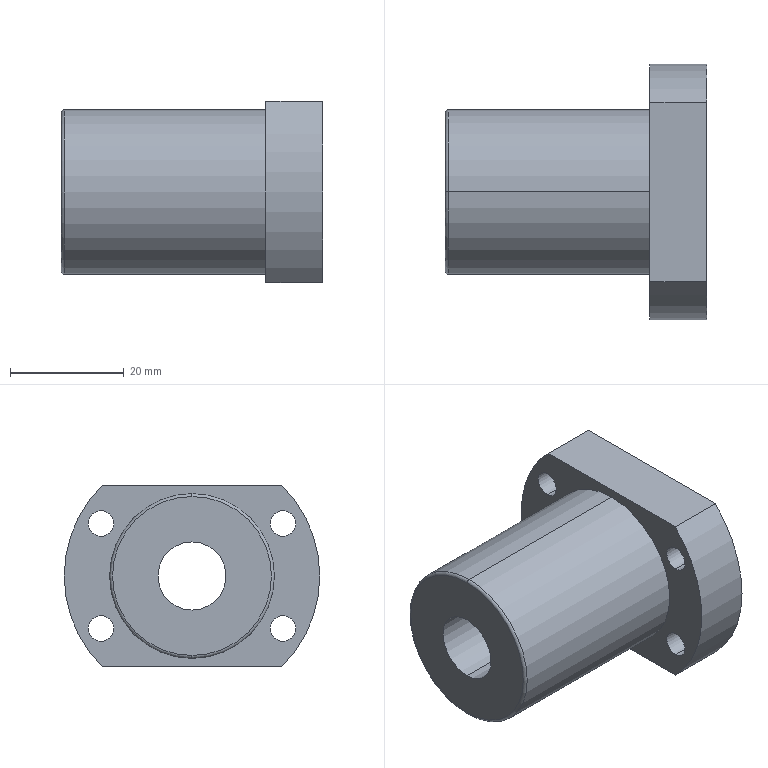Component | SolidWorks | BNK1208-2-Nut-1 | 1 solid | 21 faces | box 46 x 45 x 32 mm | volume 31007 mm3 | cylinder 14 | plane 5 | torus 2 | commonest cylinder face diameters 4.5 x8 12 x2 29 x2 45 x2
STEP:
#1=COLOUR_RGB('',0.7922,0.8196,0.9333);
#2=FILL_AREA_STYLE_COLOUR('',#1);
#3=FILL_AREA_STYLE('',(#2));
#4=SURFACE_STYLE_FILL_AREA(#3);
#5=SURFACE_SIDE_STYLE('',(#4));
#6=SURFACE_STYLE_USAGE(.BOTH.,#5);
#7=PRESENTATION_STYLE_ASSIGNMENT((#6));
#8=CARTESIAN_POINT('',(-2.212,0.7853,-0.4311));
#9=VERTEX_POINT('',#8);
#10=CARTESIAN_POINT('',(-2.212,0.7853,0.7107));
#11=VERTEX_POINT('',#10);
#12=CARTESIAN_POINT('',(-2.212,0.7853,0.1398));
#13=DIRECTION('',(1.,-0.,0.));
#14=DIRECTION('',(0.,0.,1.));
#15=AXIS2_PLACEMENT_3D('',#12,#13,#14);
#16=CIRCLE('',#15,0.5709);
#17=EDGE_CURVE('',#9,#11,#16,.T.);
#18=ORIENTED_EDGE('',*,*,#17,.F.);
#19=CARTESIAN_POINT('',(-2.232,0.7853,-0.4114));
#20=VERTEX_POINT('',#19);
#21=CARTESIAN_POINT('',(-2.212,0.7853,-0.4114));
#22=DIRECTION('',(0.,1.,-0.));
#23=DIRECTION('',(0.,0.,1.));
#24=AXIS2_PLACEMENT_3D('',#21,#22,#23);
#25=CIRCLE('',#24,0.01969);
#26=EDGE_CURVE('',#9,#20,#25,.T.);
#27=ORIENTED_EDGE('',*,*,#26,.T.);
#28=CARTESIAN_POINT('',(-2.232,0.7853,0.691));
#29=VERTEX_POINT('',#28);
#30=CARTESIAN_POINT('',(-2.232,0.7853,0.1398));
#31=DIRECTION('',(-1.,0.,-0.));
#32=DIRECTION('',(0.,0.,1.));
#33=AXIS2_PLACEMENT_3D('',#30,#31,#32);
#34=CIRCLE('',#33,0.5512);
#35=EDGE_CURVE('',#29,#20,#34,.T.);
#36=ORIENTED_EDGE('',*,*,#35,.F.);
#37=CARTESIAN_POINT('',(-2.212,0.7853,0.691));
#38=DIRECTION('',(-0.,-1.,0.));
#39=DIRECTION('',(0.,0.,-1.));
#40=AXIS2_PLACEMENT_3D('',#37,#38,#39);
#41=CIRCLE('',#40,0.01969);
#42=EDGE_CURVE('',#11,#29,#41,.T.);
#43=ORIENTED_EDGE('',*,*,#42,.F.);
#44=EDGE_LOOP('',(#18,#27,#36,#43));
#45=FACE_OUTER_BOUND('',#44,.T.);
#46=CARTESIAN_POINT('',(-2.212,0.7853,0.1398));
#47=DIRECTION('',(-1.,0.,-0.));
#48=DIRECTION('',(-0.,0.,1.));
#49=AXIS2_PLACEMENT_3D('',#46,#47,#48);
#50=TOROIDAL_SURFACE('',#49,0.5512,0.01969);
#51=ADVANCED_FACE('',(#45),#50,.T.);
#52=CARTESIAN_POINT('',(-0.8147,1.416,-0.1358));
#53=VERTEX_POINT('',#52);
#54=CARTESIAN_POINT('',(-0.8147,1.416,-0.313));
#55=VERTEX_POINT('',#54);
#56=CARTESIAN_POINT('',(-0.8147,1.416,-0.2244));
#57=DIRECTION('',(1.,-0.,0.));
#58=DIRECTION('',(0.,0.,-1.));
#59=AXIS2_PLACEMENT_3D('',#56,#57,#58);
#60=CIRCLE('',#59,0.08858);
#61=EDGE_CURVE('',#53,#55,#60,.T.);
#62=ORIENTED_EDGE('',*,*,#61,.F.);
#63=CARTESIAN_POINT('',(-0.421,1.416,-0.1358));
#64=VERTEX_POINT('',#63);
#65=CARTESIAN_POINT('',(-0.421,1.416,-0.1358));
#66=DIRECTION('',(1.,-0.,0.));
#67=VECTOR('',#66,39.37);
#68=LINE('',#65,#67);
#69=EDGE_CURVE('',#53,#64,#68,.T.);
#70=ORIENTED_EDGE('',*,*,#69,.T.);
#71=CARTESIAN_POINT('',(-0.421,1.416,-0.313));
#72=VERTEX_POINT('',#71);
#73=CARTESIAN_POINT('',(-0.421,1.416,-0.2244));
#74=DIRECTION('',(1.,-0.,0.));
#75=DIRECTION('',(0.,0.,-1.));
#76=AXIS2_PLACEMENT_3D('',#73,#74,#75);
#77=CIRCLE('',#76,0.08858);
#78=EDGE_CURVE('',#64,#72,#77,.T.);
#79=ORIENTED_EDGE('',*,*,#78,.T.);
#80=CARTESIAN_POINT('',(-0.421,1.416,-0.313));
#81=DIRECTION('',(1.,-0.,0.));
#82=VECTOR('',#81,39.37);
#83=LINE('',#80,#82);
#84=EDGE_CURVE('',#55,#72,#83,.T.);
#85=ORIENTED_EDGE('',*,*,#84,.F.);
#86=EDGE_LOOP('',(#62,#70,#79,#85));
#87=FACE_OUTER_BOUND('',#86,.T.);
#88=CARTESIAN_POINT('',(-0.421,1.416,-0.2244));
#89=DIRECTION('',(1.,-0.,0.));
#90=DIRECTION('',(0.,0.,-1.));
#91=AXIS2_PLACEMENT_3D('',#88,#89,#90);
#92=CYLINDRICAL_SURFACE('',#91,0.08858);
#93=ADVANCED_FACE('',(#87),#92,.F.);
#94=CARTESIAN_POINT('',(-0.8147,1.416,0.5925));
#95=VERTEX_POINT('',#94);
#96=CARTESIAN_POINT('',(-0.8147,1.416,0.4154));
#97=VERTEX_POINT('',#96);
#98=CARTESIAN_POINT('',(-0.8147,1.416,0.504));
#99=DIRECTION('',(1.,-0.,0.));
#100=DIRECTION('',(0.,0.,-1.));
#101=AXIS2_PLACEMENT_3D('',#98,#99,#100);
#102=CIRCLE('',#101,0.08858);
#103=EDGE_CURVE('',#95,#97,#102,.T.);
#104=ORIENTED_EDGE('',*,*,#103,.F.);
#105=CARTESIAN_POINT('',(-0.421,1.416,0.5925));
#106=VERTEX_POINT('',#105);
#107=CARTESIAN_POINT('',(-0.421,1.416,0.5925));
#108=DIRECTION('',(1.,-0.,0.));
#109=VECTOR('',#108,39.37);
#110=LINE('',#107,#109);
#111=EDGE_CURVE('',#95,#106,#110,.T.);
#112=ORIENTED_EDGE('',*,*,#111,.T.);
#113=CARTESIAN_POINT('',(-0.421,1.416,0.4154));
#114=VERTEX_POINT('',#113);
#115=CARTESIAN_POINT('',(-0.421,1.416,0.504));
#116=DIRECTION('',(1.,-0.,0.));
#117=DIRECTION('',(0.,0.,-1.));
#118=AXIS2_PLACEMENT_3D('',#115,#116,#117);
#119=CIRCLE('',#118,0.08858);
#120=EDGE_CURVE('',#106,#114,#119,.T.);
#121=ORIENTED_EDGE('',*,*,#120,.T.);
#122=CARTESIAN_POINT('',(-0.421,1.416,0.4154));
#123=DIRECTION('',(1.,-0.,0.));
#124=VECTOR('',#123,39.37);
#125=LINE('',#122,#124);
#126=EDGE_CURVE('',#97,#114,#125,.T.);
#127=ORIENTED_EDGE('',*,*,#126,.F.);
#128=EDGE_LOOP('',(#104,#112,#121,#127));
#129=FACE_OUTER_BOUND('',#128,.T.);
#130=CARTESIAN_POINT('',(-0.421,1.416,0.504));
#131=DIRECTION('',(1.,-0.,0.));
#132=DIRECTION('',(0.,0.,-1.));
#133=AXIS2_PLACEMENT_3D('',#130,#131,#132);
#134=CYLINDRICAL_SURFACE('',#133,0.08858);
#135=ADVANCED_FACE('',(#129),#134,.F.);
#136=CARTESIAN_POINT('',(-0.8147,0.1545,0.5925));
#137=VERTEX_POINT('',#136);
#138=CARTESIAN_POINT('',(-0.8147,0.1545,0.4154));
#139=VERTEX_POINT('',#138);
#140=CARTESIAN_POINT('',(-0.8147,0.1545,0.504));
#141=DIRECTION('',(1.,-0.,0.));
#142=DIRECTION('',(0.,-0.,-1.));
#143=AXIS2_PLACEMENT_3D('',#140,#141,#142);
#144=CIRCLE('',#143,0.08858);
#145=EDGE_CURVE('',#137,#139,#144,.T.);
#146=ORIENTED_EDGE('',*,*,#145,.F.);
#147=CARTESIAN_POINT('',(-0.421,0.1545,0.5925));
#148=VERTEX_POINT('',#147);
#149=CARTESIAN_POINT('',(-0.421,0.1545,0.5925));
#150=DIRECTION('',(1.,-0.,0.));
#151=VECTOR('',#150,39.37);
#152=LINE('',#149,#151);
#153=EDGE_CURVE('',#137,#148,#152,.T.);
#154=ORIENTED_EDGE('',*,*,#153,.T.);
#155=CARTESIAN_POINT('',(-0.421,0.1545,0.4154));
#156=VERTEX_POINT('',#155);
#157=CARTESIAN_POINT('',(-0.421,0.1545,0.504));
#158=DIRECTION('',(1.,-0.,0.));
#159=DIRECTION('',(0.,-0.,-1.));
#160=AXIS2_PLACEMENT_3D('',#157,#158,#159);
#161=CIRCLE('',#160,0.08858);
#162=EDGE_CURVE('',#148,#156,#161,.T.);
#163=ORIENTED_EDGE('',*,*,#162,.T.);
#164=CARTESIAN_POINT('',(-0.421,0.1545,0.4154));
#165=DIRECTION('',(1.,-0.,0.));
#166=VECTOR('',#165,39.37);
#167=LINE('',#164,#166);
#168=EDGE_CURVE('',#139,#156,#167,.T.);
#169=ORIENTED_EDGE('',*,*,#168,.F.);
#170=EDGE_LOOP('',(#146,#154,#163,#169));
#171=FACE_OUTER_BOUND('',#170,.T.);
#172=CARTESIAN_POINT('',(-0.421,0.1545,0.504));
#173=DIRECTION('',(1.,-0.,0.));
#174=DIRECTION('',(0.,-0.,-1.));
#175=AXIS2_PLACEMENT_3D('',#172,#173,#174);
#176=CYLINDRICAL_SURFACE('',#175,0.08858);
#177=ADVANCED_FACE('',(#171),#176,.F.);
#178=CARTESIAN_POINT('',(-0.8147,0.1545,-0.1358));
#179=VERTEX_POINT('',#178);
#180=CARTESIAN_POINT('',(-0.8147,0.1545,-0.313));
#181=VERTEX_POINT('',#180);
#182=CARTESIAN_POINT('',(-0.8147,0.1545,-0.2244));
#183=DIRECTION('',(1.,-0.,0.));
#184=DIRECTION('',(0.,-0.,-1.));
#185=AXIS2_PLACEMENT_3D('',#182,#183,#184);
#186=CIRCLE('',#185,0.08858);
#187=EDGE_CURVE('',#179,#181,#186,.T.);
#188=ORIENTED_EDGE('',*,*,#187,.F.);
#189=CARTESIAN_POINT('',(-0.421,0.1545,-0.1358));
#190=VERTEX_POINT('',#189);
#191=CARTESIAN_POINT('',(-0.421,0.1545,-0.1358));
#192=DIRECTION('',(1.,-0.,0.));
#193=VECTOR('',#192,39.37);
#194=LINE('',#191,#193);
#195=EDGE_CURVE('',#179,#190,#194,.T.);
#196=ORIENTED_EDGE('',*,*,#195,.T.);
#197=CARTESIAN_POINT('',(-0.421,0.1545,-0.313));
#198=VERTEX_POINT('',#197);
#199=CARTESIAN_POINT('',(-0.421,0.1545,-0.2244));
#200=DIRECTION('',(1.,-0.,0.));
#201=DIRECTION('',(0.,-0.,-1.));
#202=AXIS2_PLACEMENT_3D('',#199,#200,#201);
#203=CIRCLE('',#202,0.08858);
#204=EDGE_CURVE('',#190,#198,#203,.T.);
#205=ORIENTED_EDGE('',*,*,#204,.T.);
#206=CARTESIAN_POINT('',(-0.421,0.1545,-0.313));
#207=DIRECTION('',(1.,-0.,0.));
#208=VECTOR('',#207,39.37);
#209=LINE('',#206,#208);
#210=EDGE_CURVE('',#181,#198,#209,.T.);
#211=ORIENTED_EDGE('',*,*,#210,.F.);
#212=EDGE_LOOP('',(#188,#196,#205,#211));
#213=FACE_OUTER_BOUND('',#212,.T.);
#214=CARTESIAN_POINT('',(-0.421,0.1545,-0.2244));
#215=DIRECTION('',(1.,-0.,0.));
#216=DIRECTION('',(0.,-0.,-1.));
#217=AXIS2_PLACEMENT_3D('',#214,#215,#216);
#218=CYLINDRICAL_SURFACE('',#217,0.08858);
#219=ADVANCED_FACE('',(#213),#218,.F.);
#220=CARTESIAN_POINT('',(-2.232,0.7853,-0.09643));
#221=VERTEX_POINT('',#220);
#222=CARTESIAN_POINT('',(-2.232,0.7853,0.376));
#223=VERTEX_POINT('',#222);
#224=CARTESIAN_POINT('',(-2.232,0.7853,0.1398));
#225=DIRECTION('',(-1.,0.,-0.));
#226=DIRECTION('',(0.,0.,1.));
#227=AXIS2_PLACEMENT_3D('',#224,#225,#226);
#228=CIRCLE('',#227,0.2362);
#229=EDGE_CURVE('',#221,#223,#228,.T.);
#230=ORIENTED_EDGE('',*,*,#229,.T.);
#231=CARTESIAN_POINT('',(-0.421,0.7853,0.376));
#232=VERTEX_POINT('',#231);
#233=CARTESIAN_POINT('',(-2.39,0.7853,0.376));
#234=DIRECTION('',(1.,-0.,0.));
#235=VECTOR('',#234,39.37);
#236=LINE('',#233,#235);
#237=EDGE_CURVE('',#223,#232,#236,.T.);
#238=ORIENTED_EDGE('',*,*,#237,.T.);
#239=CARTESIAN_POINT('',(-0.421,0.7853,-0.09643));
#240=VERTEX_POINT('',#239);
#241=CARTESIAN_POINT('',(-0.421,0.7853,0.1398));
#242=DIRECTION('',(1.,-0.,0.));
#243=DIRECTION('',(0.,-0.,-1.));
#244=AXIS2_PLACEMENT_3D('',#241,#242,#243);
#245=CIRCLE('',#244,0.2362);
#246=EDGE_CURVE('',#232,#240,#245,.T.);
#247=ORIENTED_EDGE('',*,*,#246,.T.);
#248=CARTESIAN_POINT('',(-2.39,0.7853,-0.09643));
#249=DIRECTION('',(1.,-0.,0.));
#250=VECTOR('',#249,39.37);
#251=LINE('',#248,#250);
#252=EDGE_CURVE('',#221,#240,#251,.T.);
#253=ORIENTED_EDGE('',*,*,#252,.F.);
#254=EDGE_LOOP('',(#230,#238,#247,#253));
#255=FACE_OUTER_BOUND('',#254,.T.);
#256=CARTESIAN_POINT('',(-2.39,0.7853,0.1398));
#257=DIRECTION('',(1.,-0.,0.));
#258=DIRECTION('',(0.,-0.,-1.));
#259=AXIS2_PLACEMENT_3D('',#256,#257,#258);
#260=CYLINDRICAL_SURFACE('',#259,0.2362);
#261=ADVANCED_FACE('',(#255),#260,.F.);
#262=ORIENTED_EDGE('',*,*,#17,.T.);
#263=CARTESIAN_POINT('',(-0.8147,0.7853,0.7107));
#264=VERTEX_POINT('',#263);
#265=CARTESIAN_POINT('',(-2.232,0.7853,0.7107));
#266=DIRECTION('',(1.,-0.,0.));
#267=VECTOR('',#266,39.37);
#268=LINE('',#265,#267);
#269=EDGE_CURVE('',#11,#264,#268,.T.);
#270=ORIENTED_EDGE('',*,*,#269,.T.);
#271=CARTESIAN_POINT('',(-0.8147,0.7853,-0.4311));
#272=VERTEX_POINT('',#271);
#273=CARTESIAN_POINT('',(-0.8147,0.7853,0.1398));
#274=DIRECTION('',(1.,-0.,0.));
#275=DIRECTION('',(0.,-0.,-1.));
#276=AXIS2_PLACEMENT_3D('',#273,#274,#275);
#277=CIRCLE('',#276,0.5709);
#278=EDGE_CURVE('',#272,#264,#277,.T.);
#279=ORIENTED_EDGE('',*,*,#278,.F.);
#280=CARTESIAN_POINT('',(-2.232,0.7853,-0.4311));
#281=DIRECTION('',(1.,-0.,0.));
#282=VECTOR('',#281,39.37);
#283=LINE('',#280,#282);
#284=EDGE_CURVE('',#9,#272,#283,.T.);
#285=ORIENTED_EDGE('',*,*,#284,.F.);
#286=EDGE_LOOP('',(#262,#270,#279,#285));
#287=FACE_OUTER_BOUND('',#286,.T.);
#288=CARTESIAN_POINT('',(-2.232,0.7853,0.1398));
#289=DIRECTION('',(1.,-0.,0.));
#290=DIRECTION('',(0.,-0.,-1.));
#291=AXIS2_PLACEMENT_3D('',#288,#289,#290);
#292=CYLINDRICAL_SURFACE('',#291,0.5709);
#293=ADVANCED_FACE('',(#287),#292,.T.);
#294=CARTESIAN_POINT('',(-0.421,0.1624,0.7697));
#295=VERTEX_POINT('',#294);
#296=CARTESIAN_POINT('',(-0.421,0.1624,-0.4901));
#297=VERTEX_POINT('',#296);
#298=CARTESIAN_POINT('',(-0.421,0.7853,0.1398));
#299=DIRECTION('',(1.,-0.,0.));
#300=DIRECTION('',(0.,-0.,-1.));
#301=AXIS2_PLACEMENT_3D('',#298,#299,#300);
#302=CIRCLE('',#301,0.8858);
#303=EDGE_CURVE('',#295,#297,#302,.T.);
#304=ORIENTED_EDGE('',*,*,#303,.F.);
#305=CARTESIAN_POINT('',(-0.8147,0.1624,0.7697));
#306=VERTEX_POINT('',#305);
#307=CARTESIAN_POINT('',(-2.39,0.1624,0.7697));
#308=DIRECTION('',(1.,-0.,0.));
#309=VECTOR('',#308,39.37);
#310=LINE('',#307,#309);
#311=EDGE_CURVE('',#306,#295,#310,.T.);
#312=ORIENTED_EDGE('',*,*,#311,.F.);
#313=CARTESIAN_POINT('',(-0.8147,0.1624,-0.4901));
#314=VERTEX_POINT('',#313);
#315=CARTESIAN_POINT('',(-0.8147,0.7853,0.1398));
#316=DIRECTION('',(1.,-0.,0.));
#317=DIRECTION('',(0.,-0.,-1.));
#318=AXIS2_PLACEMENT_3D('',#315,#316,#317);
#319=CIRCLE('',#318,0.8858);
#320=EDGE_CURVE('',#306,#314,#319,.T.);
#321=ORIENTED_EDGE('',*,*,#320,.T.);
#322=CARTESIAN_POINT('',(-2.39,0.1624,-0.4901));
#323=DIRECTION('',(1.,-0.,0.));
#324=VECTOR('',#323,39.37);
#325=LINE('',#322,#324);
#326=EDGE_CURVE('',#314,#297,#325,.T.);
#327=ORIENTED_EDGE('',*,*,#326,.T.);
#328=EDGE_LOOP('',(#304,#312,#321,#327));
#329=FACE_OUTER_BOUND('',#328,.T.);
#330=CARTESIAN_POINT('',(-0.421,0.7853,0.1398));
#331=DIRECTION('',(-1.,0.,-0.));
#332=DIRECTION('',(0.,0.,1.));
#333=AXIS2_PLACEMENT_3D('',#330,#331,#332);
#334=CYLINDRICAL_SURFACE('',#333,0.8858);
#335=ADVANCED_FACE('',(#329),#334,.T.);
#336=ORIENTED_EDGE('',*,*,#269,.F.);
#337=CARTESIAN_POINT('',(-2.212,0.7853,0.1398));
#338=DIRECTION('',(1.,-0.,0.));
#339=DIRECTION('',(0.,0.,1.));
#340=AXIS2_PLACEMENT_3D('',#337,#338,#339);
#341=CIRCLE('',#340,0.5709);
#342=EDGE_CURVE('',#11,#9,#341,.T.);
#343=ORIENTED_EDGE('',*,*,#342,.T.);
#344=ORIENTED_EDGE('',*,*,#284,.T.);
#345=CARTESIAN_POINT('',(-0.8147,0.7853,0.1398));
#346=DIRECTION('',(1.,-0.,0.));
#347=DIRECTION('',(0.,-0.,-1.));
#348=AXIS2_PLACEMENT_3D('',#345,#346,#347);
#349=CIRCLE('',#348,0.5709);
#350=EDGE_CURVE('',#264,#272,#349,.T.);
#351=ORIENTED_EDGE('',*,*,#350,.F.);
#352=EDGE_LOOP('',(#336,#343,#344,#351));
#353=FACE_OUTER_BOUND('',#352,.T.);
#354=CARTESIAN_POINT('',(-2.232,0.7853,0.1398));
#355=DIRECTION('',(1.,-0.,0.));
#356=DIRECTION('',(0.,-0.,-1.));
#357=AXIS2_PLACEMENT_3D('',#354,#355,#356);
#358=CYLINDRICAL_SURFACE('',#357,0.5709);
#359=ADVANCED_FACE('',(#353),#358,.T.);
#360=ORIENTED_EDGE('',*,*,#35,.T.);
#361=CARTESIAN_POINT('',(-2.232,0.7853,0.1398));
#362=DIRECTION('',(-1.,0.,-0.));
#363=DIRECTION('',(0.,0.,1.));
#364=AXIS2_PLACEMENT_3D('',#361,#362,#363);
#365=CIRCLE('',#364,0.5512);
#366=EDGE_CURVE('',#20,#29,#365,.T.);
#367=ORIENTED_EDGE('',*,*,#366,.T.);
#368=EDGE_LOOP('',(#360,#367));
#369=FACE_OUTER_BOUND('',#368,.T.);
#370=ORIENTED_EDGE('',*,*,#229,.F.);
#371=CARTESIAN_POINT('',(-2.232,0.7853,0.1398));
#372=DIRECTION('',(-1.,0.,-0.));
#373=DIRECTION('',(0.,0.,1.));
#374=AXIS2_PLACEMENT_3D('',#371,#372,#373);
#375=CIRCLE('',#374,0.2362);
#376=EDGE_CURVE('',#223,#221,#375,.T.);
#377=ORIENTED_EDGE('',*,*,#376,.F.);
#378=EDGE_LOOP('',(#370,#377));
#379=FACE_BOUND('',#378,.T.);
#380=CARTESIAN_POINT('',(-2.232,0.7853,0.1398));
#381=DIRECTION('',(-1.,0.,-0.));
#382=DIRECTION('',(-0.,0.,1.));
#383=AXIS2_PLACEMENT_3D('',#380,#381,#382);
#384=PLANE('',#383);
#385=ADVANCED_FACE('',(#369,#379),#384,.T.);
#386=CARTESIAN_POINT('',(-0.8147,1.416,-0.2244));
#387=DIRECTION('',(1.,-0.,0.));
#388=DIRECTION('',(0.,0.,-1.));
#389=AXIS2_PLACEMENT_3D('',#386,#387,#388);
#390=CIRCLE('',#389,0.08858);
#391=EDGE_CURVE('',#55,#53,#390,.T.);
#392=ORIENTED_EDGE('',*,*,#391,.T.);
#393=ORIENTED_EDGE('',*,*,#61,.T.);
#394=EDGE_LOOP('',(#392,#393));
#395=FACE_BOUND('',#394,.T.);
#396=CARTESIAN_POINT('',(-0.8147,1.416,0.504));
#397=DIRECTION('',(1.,-0.,0.));
#398=DIRECTION('',(0.,0.,-1.));
#399=AXIS2_PLACEMENT_3D('',#396,#397,#398);
#400=CIRCLE('',#399,0.08858);
#401=EDGE_CURVE('',#97,#95,#400,.T.);
#402=ORIENTED_EDGE('',*,*,#401,.T.);
#403=ORIENTED_EDGE('',*,*,#103,.T.);
#404=EDGE_LOOP('',(#402,#403));
#405=FACE_BOUND('',#404,.T.);
#406=CARTESIAN_POINT('',(-0.8147,0.1545,0.504));
#407=DIRECTION('',(1.,-0.,0.));
#408=DIRECTION('',(0.,-0.,-1.));
#409=AXIS2_PLACEMENT_3D('',#406,#407,#408);
#410=CIRCLE('',#409,0.08858);
#411=EDGE_CURVE('',#139,#137,#410,.T.);
#412=ORIENTED_EDGE('',*,*,#411,.T.);
#413=ORIENTED_EDGE('',*,*,#145,.T.);
#414=EDGE_LOOP('',(#412,#413));
#415=FACE_BOUND('',#414,.T.);
#416=CARTESIAN_POINT('',(-0.8147,0.1545,-0.2244));
#417=DIRECTION('',(1.,-0.,0.));
#418=DIRECTION('',(0.,-0.,-1.));
#419=AXIS2_PLACEMENT_3D('',#416,#417,#418);
#420=CIRCLE('',#419,0.08858);
#421=EDGE_CURVE('',#181,#179,#420,.T.);
#422=ORIENTED_EDGE('',*,*,#421,.T.);
#423=ORIENTED_EDGE('',*,*,#187,.T.);
#424=EDGE_LOOP('',(#422,#423));
#425=FACE_BOUND('',#424,.T.);
#426=ORIENTED_EDGE('',*,*,#320,.F.);
#427=CARTESIAN_POINT('',(-0.8147,1.408,0.7697));
#428=VERTEX_POINT('',#427);
#429=CARTESIAN_POINT('',(-0.8147,0.7853,0.7697));
#430=DIRECTION('',(0.,1.,-0.));
#431=VECTOR('',#430,39.37);
#432=LINE('',#429,#431);
#433=EDGE_CURVE('',#306,#428,#432,.T.);
#434=ORIENTED_EDGE('',*,*,#433,.T.);
#435=CARTESIAN_POINT('',(-0.8147,1.408,-0.4901));
#436=VERTEX_POINT('',#435);
#437=CARTESIAN_POINT('',(-0.8147,0.7853,0.1398));
#438=DIRECTION('',(1.,-0.,0.));
#439=DIRECTION('',(0.,-0.,-1.));
#440=AXIS2_PLACEMENT_3D('',#437,#438,#439);
#441=CIRCLE('',#440,0.8858);
#442=EDGE_CURVE('',#436,#428,#441,.T.);
#443=ORIENTED_EDGE('',*,*,#442,.F.);
#444=CARTESIAN_POINT('',(-0.8147,0.7853,-0.4901));
#445=DIRECTION('',(-0.,-1.,0.));
#446=VECTOR('',#445,39.37);
#447=LINE('',#444,#446);
#448=EDGE_CURVE('',#436,#314,#447,.T.);
#449=ORIENTED_EDGE('',*,*,#448,.T.);
#450=EDGE_LOOP('',(#426,#434,#443,#449));
#451=FACE_OUTER_BOUND('',#450,.T.);
#452=ORIENTED_EDGE('',*,*,#278,.T.);
#453=ORIENTED_EDGE('',*,*,#350,.T.);
#454=EDGE_LOOP('',(#452,#453));
#455=FACE_BOUND('',#454,.T.);
#456=CARTESIAN_POINT('',(-0.8147,0.7853,0.1398));
#457=DIRECTION('',(1.,-0.,0.));
#458=DIRECTION('',(0.,-0.,-1.));
#459=AXIS2_PLACEMENT_3D('',#456,#457,#458);
#460=PLANE('',#459);
#461=ADVANCED_FACE('',(#395,#405,#415,#425,#451,#455),#460,.F.);
#462=ORIENTED_EDGE('',*,*,#442,.T.);
#463=CARTESIAN_POINT('',(-0.421,1.408,0.7697));
#464=VERTEX_POINT('',#463);
#465=CARTESIAN_POINT('',(-2.39,1.408,0.7697));
#466=DIRECTION('',(1.,-0.,0.));
#467=VECTOR('',#466,39.37);
#468=LINE('',#465,#467);
#469=EDGE_CURVE('',#428,#464,#468,.T.);
#470=ORIENTED_EDGE('',*,*,#469,.T.);
#471=CARTESIAN_POINT('',(-0.421,1.408,-0.4901));
#472=VERTEX_POINT('',#471);
#473=CARTESIAN_POINT('',(-0.421,0.7853,0.1398));
#474=DIRECTION('',(1.,-0.,0.));
#475=DIRECTION('',(0.,-0.,-1.));
#476=AXIS2_PLACEMENT_3D('',#473,#474,#475);
#477=CIRCLE('',#476,0.8858);
#478=EDGE_CURVE('',#472,#464,#477,.T.);
#479=ORIENTED_EDGE('',*,*,#478,.F.);
#480=CARTESIAN_POINT('',(-2.39,1.408,-0.4901));
#481=DIRECTION('',(1.,-0.,0.));
#482=VECTOR('',#481,39.37);
#483=LINE('',#480,#482);
#484=EDGE_CURVE('',#436,#472,#483,.T.);
#485=ORIENTED_EDGE('',*,*,#484,.F.);
#486=EDGE_LOOP('',(#462,#470,#479,#485));
#487=FACE_OUTER_BOUND('',#486,.T.);
#488=CARTESIAN_POINT('',(-0.421,0.7853,0.1398));
#489=DIRECTION('',(-1.,0.,-0.));
#490=DIRECTION('',(0.,0.,1.));
#491=AXIS2_PLACEMENT_3D('',#488,#489,#490);
#492=CYLINDRICAL_SURFACE('',#491,0.8858);
#493=ADVANCED_FACE('',(#487),#492,.T.);
#494=CARTESIAN_POINT('',(-0.421,1.416,-0.2244));
#495=DIRECTION('',(1.,-0.,0.));
#496=DIRECTION('',(0.,0.,-1.));
#497=AXIS2_PLACEMENT_3D('',#494,#495,#496);
#498=CIRCLE('',#497,0.08858);
#499=EDGE_CURVE('',#72,#64,#498,.T.);
#500=ORIENTED_EDGE('',*,*,#499,.F.);
#501=ORIENTED_EDGE('',*,*,#78,.F.);
#502=EDGE_LOOP('',(#500,#501));
#503=FACE_BOUND('',#502,.T.);
#504=CARTESIAN_POINT('',(-0.421,1.416,0.504));
#505=DIRECTION('',(1.,-0.,0.));
#506=DIRECTION('',(0.,0.,-1.));
#507=AXIS2_PLACEMENT_3D('',#504,#505,#506);
#508=CIRCLE('',#507,0.08858);
#509=EDGE_CURVE('',#114,#106,#508,.T.);
#510=ORIENTED_EDGE('',*,*,#509,.F.);
#511=ORIENTED_EDGE('',*,*,#120,.F.);
#512=EDGE_LOOP('',(#510,#511));
#513=FACE_BOUND('',#512,.T.);
#514=CARTESIAN_POINT('',(-0.421,0.1545,0.504));
#515=DIRECTION('',(1.,-0.,0.));
#516=DIRECTION('',(0.,-0.,-1.));
#517=AXIS2_PLACEMENT_3D('',#514,#515,#516);
#518=CIRCLE('',#517,0.08858);
#519=EDGE_CURVE('',#156,#148,#518,.T.);
#520=ORIENTED_EDGE('',*,*,#519,.F.);
#521=ORIENTED_EDGE('',*,*,#162,.F.);
#522=EDGE_LOOP('',(#520,#521));
#523=FACE_BOUND('',#522,.T.);
#524=CARTESIAN_POINT('',(-0.421,0.1545,-0.2244));
#525=DIRECTION('',(1.,-0.,0.));
#526=DIRECTION('',(0.,-0.,-1.));
#527=AXIS2_PLACEMENT_3D('',#524,#525,#526);
#528=CIRCLE('',#527,0.08858);
#529=EDGE_CURVE('',#198,#190,#528,.T.);
#530=ORIENTED_EDGE('',*,*,#529,.F.);
#531=ORIENTED_EDGE('',*,*,#204,.F.);
#532=EDGE_LOOP('',(#530,#531));
#533=FACE_BOUND('',#532,.T.);
#534=CARTESIAN_POINT('',(-0.421,0.7853,0.1398));
#535=DIRECTION('',(1.,-0.,0.));
#536=DIRECTION('',(0.,-0.,-1.));
#537=AXIS2_PLACEMENT_3D('',#534,#535,#536);
#538=CIRCLE('',#537,0.2362);
#539=EDGE_CURVE('',#240,#232,#538,.T.);
#540=ORIENTED_EDGE('',*,*,#539,.F.);
#541=ORIENTED_EDGE('',*,*,#246,.F.);
#542=EDGE_LOOP('',(#540,#541));
#543=FACE_BOUND('',#542,.T.);
#544=CARTESIAN_POINT('',(-0.421,1.408,0.7697));
#545=DIRECTION('',(0.,1.,-0.));
#546=VECTOR('',#545,39.37);
#547=LINE('',#544,#546);
#548=EDGE_CURVE('',#295,#464,#547,.T.);
#549=ORIENTED_EDGE('',*,*,#548,.F.);
#550=ORIENTED_EDGE('',*,*,#303,.T.);
#551=CARTESIAN_POINT('',(-0.421,1.408,-0.4901));
#552=DIRECTION('',(-0.,-1.,0.));
#553=VECTOR('',#552,39.37);
#554=LINE('',#551,#553);
#555=EDGE_CURVE('',#472,#297,#554,.T.);
#556=ORIENTED_EDGE('',*,*,#555,.F.);
#557=ORIENTED_EDGE('',*,*,#478,.T.);
#558=EDGE_LOOP('',(#549,#550,#556,#557));
#559=FACE_OUTER_BOUND('',#558,.T.);
#560=CARTESIAN_POINT('',(-0.421,0.7853,0.1398));
#561=DIRECTION('',(1.,-0.,0.));
#562=DIRECTION('',(0.,-0.,-1.));
#563=AXIS2_PLACEMENT_3D('',#560,#561,#562);
#564=PLANE('',#563);
#565=ADVANCED_FACE('',(#503,#513,#523,#533,#543,#559),#564,.T.);
#566=ORIENTED_EDGE('',*,*,#484,.T.);
#567=ORIENTED_EDGE('',*,*,#555,.T.);
#568=ORIENTED_EDGE('',*,*,#326,.F.);
#569=ORIENTED_EDGE('',*,*,#448,.F.);
#570=EDGE_LOOP('',(#566,#567,#568,#569));
#571=FACE_OUTER_BOUND('',#570,.T.);
#572=CARTESIAN_POINT('',(-2.39,1.408,-0.4901));
#573=DIRECTION('',(-0.,0.,1.));
#574=DIRECTION('',(1.,-0.,0.));
#575=AXIS2_PLACEMENT_3D('',#572,#573,#574);
#576=PLANE('',#575);
#577=ADVANCED_FACE('',(#571),#576,.F.);
#578=ORIENTED_EDGE('',*,*,#311,.T.);
#579=ORIENTED_EDGE('',*,*,#548,.T.);
#580=ORIENTED_EDGE('',*,*,#469,.F.);
#581=ORIENTED_EDGE('',*,*,#433,.F.);
#582=EDGE_LOOP('',(#578,#579,#580,#581));
#583=FACE_OUTER_BOUND('',#582,.T.);
#584=CARTESIAN_POINT('',(-2.39,1.408,0.7697));
#585=DIRECTION('',(0.,-0.,-1.));
#586=DIRECTION('',(-1.,0.,-0.));
#587=AXIS2_PLACEMENT_3D('',#584,#585,#586);
#588=PLANE('',#587);
#589=ADVANCED_FACE('',(#583),#588,.F.);
#590=ORIENTED_EDGE('',*,*,#237,.F.);
#591=ORIENTED_EDGE('',*,*,#376,.T.);
#592=ORIENTED_EDGE('',*,*,#252,.T.);
#593=ORIENTED_EDGE('',*,*,#539,.T.);
#594=EDGE_LOOP('',(#590,#591,#592,#593));
#595=FACE_OUTER_BOUND('',#594,.T.);
#596=CARTESIAN_POINT('',(-2.39,0.7853,0.1398));
#597=DIRECTION('',(1.,-0.,0.));
#598=DIRECTION('',(0.,-0.,-1.));
#599=AXIS2_PLACEMENT_3D('',#596,#597,#598);
#600=CYLINDRICAL_SURFACE('',#599,0.2362);
#601=ADVANCED_FACE('',(#595),#600,.F.);
#602=ORIENTED_EDGE('',*,*,#195,.F.);
#603=ORIENTED_EDGE('',*,*,#421,.F.);
#604=ORIENTED_EDGE('',*,*,#210,.T.);
#605=ORIENTED_EDGE('',*,*,#529,.T.);
#606=EDGE_LOOP('',(#602,#603,#604,#605));
#607=FACE_OUTER_BOUND('',#606,.T.);
#608=CARTESIAN_POINT('',(-0.421,0.1545,-0.2244));
#609=DIRECTION('',(1.,-0.,0.));
#610=DIRECTION('',(0.,-0.,-1.));
#611=AXIS2_PLACEMENT_3D('',#608,#609,#610);
#612=CYLINDRICAL_SURFACE('',#611,0.08858);
#613=ADVANCED_FACE('',(#607),#612,.F.);
#614=ORIENTED_EDGE('',*,*,#153,.F.);
#615=ORIENTED_EDGE('',*,*,#411,.F.);
#616=ORIENTED_EDGE('',*,*,#168,.T.);
#617=ORIENTED_EDGE('',*,*,#519,.T.);
#618=EDGE_LOOP('',(#614,#615,#616,#617));
#619=FACE_OUTER_BOUND('',#618,.T.);
#620=CARTESIAN_POINT('',(-0.421,0.1545,0.504));
#621=DIRECTION('',(1.,-0.,0.));
#622=DIRECTION('',(0.,-0.,-1.));
#623=AXIS2_PLACEMENT_3D('',#620,#621,#622);
#624=CYLINDRICAL_SURFACE('',#623,0.08858);
#625=ADVANCED_FACE('',(#619),#624,.F.);
#626=ORIENTED_EDGE('',*,*,#111,.F.);
#627=ORIENTED_EDGE('',*,*,#401,.F.);
#628=ORIENTED_EDGE('',*,*,#126,.T.);
#629=ORIENTED_EDGE('',*,*,#509,.T.);
#630=EDGE_LOOP('',(#626,#627,#628,#629));
#631=FACE_OUTER_BOUND('',#630,.T.);
#632=CARTESIAN_POINT('',(-0.421,1.416,0.504));
#633=DIRECTION('',(1.,-0.,0.));
#634=DIRECTION('',(0.,0.,-1.));
#635=AXIS2_PLACEMENT_3D('',#632,#633,#634);
#636=CYLINDRICAL_SURFACE('',#635,0.08858);
#637=ADVANCED_FACE('',(#631),#636,.F.);
#638=ORIENTED_EDGE('',*,*,#69,.F.);
#639=ORIENTED_EDGE('',*,*,#391,.F.);
#640=ORIENTED_EDGE('',*,*,#84,.T.);
#641=ORIENTED_EDGE('',*,*,#499,.T.);
#642=EDGE_LOOP('',(#638,#639,#640,#641));
#643=FACE_OUTER_BOUND('',#642,.T.);
#644=CARTESIAN_POINT('',(-0.421,1.416,-0.2244));
#645=DIRECTION('',(1.,-0.,0.));
#646=DIRECTION('',(0.,0.,-1.));
#647=AXIS2_PLACEMENT_3D('',#644,#645,#646);
#648=CYLINDRICAL_SURFACE('',#647,0.08858);
#649=ADVANCED_FACE('',(#643),#648,.F.);
#650=ORIENTED_EDGE('',*,*,#26,.F.);
#651=ORIENTED_EDGE('',*,*,#342,.F.);
#652=ORIENTED_EDGE('',*,*,#42,.T.);
#653=ORIENTED_EDGE('',*,*,#366,.F.);
#654=EDGE_LOOP('',(#650,#651,#652,#653));
#655=FACE_OUTER_BOUND('',#654,.T.);
#656=CARTESIAN_POINT('',(-2.212,0.7853,0.1398));
#657=DIRECTION('',(-1.,0.,-0.));
#658=DIRECTION('',(-0.,0.,1.));
#659=AXIS2_PLACEMENT_3D('',#656,#657,#658);
#660=TOROIDAL_SURFACE('',#659,0.5512,0.01969);
#661=ADVANCED_FACE('',(#655),#660,.T.);
#662=CLOSED_SHELL('',(#51,#93,#135,#177,#219,#261,#293,#335,#359,#385,#461,#493,#565,#577,#589,#601,#613,#625,#637,#649,#661));
#663=MANIFOLD_SOLID_BREP('',#662);
#664=STYLED_ITEM('',(#7),#663);
#665=(LENGTH_UNIT()NAMED_UNIT(*)SI_UNIT($,.METRE.));
#666=LENGTH_MEASURE_WITH_UNIT(LENGTH_MEASURE(0.0254),#665);
#667=DIMENSIONAL_EXPONENTS(1.,0.,0.,0.,0.,0.,0.);
#668=(CONVERSION_BASED_UNIT('',#666)LENGTH_UNIT()NAMED_UNIT(#667));
#669=UNCERTAINTY_MEASURE_WITH_UNIT(LENGTH_MEASURE(0.00001),#668,'','');
#670=(NAMED_UNIT(*)PLANE_ANGLE_UNIT()SI_UNIT($,.RADIAN.));
#671=(NAMED_UNIT(*)SI_UNIT($,.STERADIAN.)SOLID_ANGLE_UNIT());
#672=(GEOMETRIC_REPRESENTATION_CONTEXT(3)GLOBAL_UNCERTAINTY_ASSIGNED_CONTEXT((#669))GLOBAL_UNIT_ASSIGNED_CONTEXT((#668,#670,#671))REPRESENTATION_CONTEXT('',''));
#673=MECHANICAL_DESIGN_GEOMETRIC_PRESENTATION_REPRESENTATION('',(#664),#672);
#674=PRESENTATION_LAYER_ASSIGNMENT('','',(#664));
#675=CARTESIAN_POINT('',(0.,0.,0.));
#676=DIRECTION('',(0.,0.,1.));
#677=DIRECTION('',(1.,0.,0.));
#678=AXIS2_PLACEMENT_3D('',#675,#676,#677);
#679=(LENGTH_UNIT()NAMED_UNIT(*)SI_UNIT($,.METRE.));
#680=LENGTH_MEASURE_WITH_UNIT(LENGTH_MEASURE(0.0254),#679);
#681=DIMENSIONAL_EXPONENTS(1.,0.,0.,0.,0.,0.,0.);
#682=(CONVERSION_BASED_UNIT('',#680)LENGTH_UNIT()NAMED_UNIT(#681));
#683=UNCERTAINTY_MEASURE_WITH_UNIT(LENGTH_MEASURE(0.00001),#682,'','');
#684=(NAMED_UNIT(*)PLANE_ANGLE_UNIT()SI_UNIT($,.RADIAN.));
#685=(NAMED_UNIT(*)SI_UNIT($,.STERADIAN.)SOLID_ANGLE_UNIT());
#686=(GEOMETRIC_REPRESENTATION_CONTEXT(3)GLOBAL_UNCERTAINTY_ASSIGNED_CONTEXT((#683))GLOBAL_UNIT_ASSIGNED_CONTEXT((#682,#684,#685))REPRESENTATION_CONTEXT('',''));
#687=ADVANCED_BREP_SHAPE_REPRESENTATION('',(#663,#678),#686);